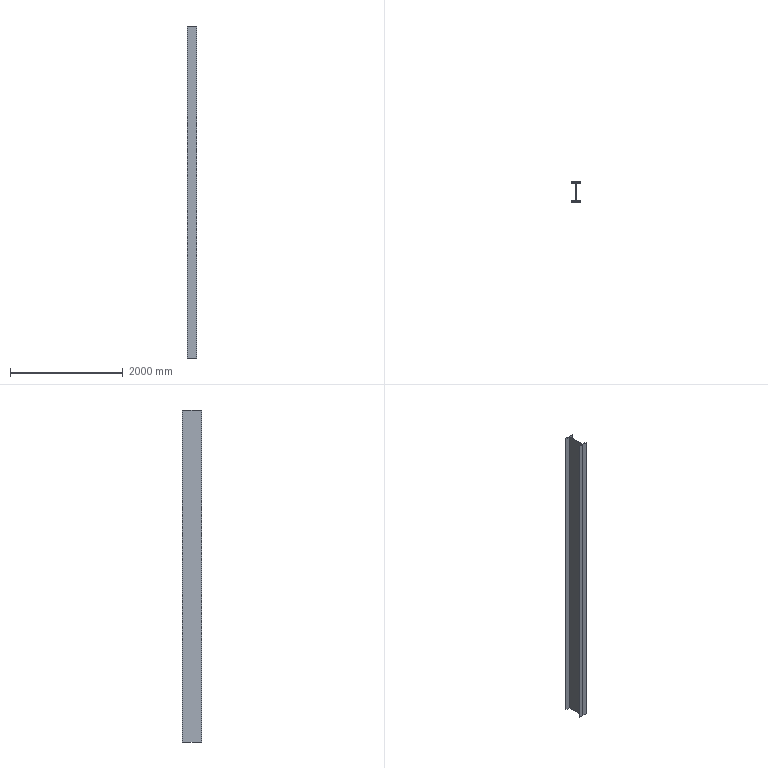Component | NX | ZHIJIA3 | 1 solid | 14 faces | box 175 x 350 x 5900 mm | volume 40120000 mm3 | plane 14
STEP:
#1=CARTESIAN_POINT('',(0.,0.,0.));
#2=DIRECTION('',(0.,0.,1.));
#3=DIRECTION('',(1.,0.,0.));
#4=AXIS2_PLACEMENT_3D('',#1,#2,#3);
#5=CARTESIAN_POINT('',(2412.5,-2965.,800.));
#6=VERTEX_POINT('',#5);
#7=CARTESIAN_POINT('',(2412.5,-2975.,800.));
#8=VERTEX_POINT('',#7);
#9=CARTESIAN_POINT('',(2412.5,-2965.,800.));
#10=DIRECTION('',(-0.,-1.,0.));
#11=VECTOR('',#10,1.);
#12=LINE('',#9,#11);
#13=CARTESIAN_POINT('',(2412.5,-2965.,6700.));
#14=DIRECTION('',(1.,-0.,0.));
#15=DIRECTION('',(0.,1.,0.));
#16=AXIS2_PLACEMENT_3D('',#13,#14,#15);
#17=PLANE('',#16);
#18=CARTESIAN_POINT('',(0.,-5900.));
#19=DIRECTION('',(-1.,0.));
#20=VECTOR('',#19,1.);
#21=LINE('',#18,#20);
#22=(GEOMETRIC_REPRESENTATION_CONTEXT(2)PARAMETRIC_REPRESENTATION_CONTEXT()REPRESENTATION_CONTEXT('',''));
#23=DEFINITIONAL_REPRESENTATION('',(#21),#22);
#24=PCURVE('',#17,#23);
#25=CARTESIAN_POINT('',(2412.5,-2975.,800.));
#26=DIRECTION('',(0.,0.,1.));
#27=DIRECTION('',(1.,0.,0.));
#28=AXIS2_PLACEMENT_3D('',#25,#26,#27);
#29=PLANE('',#28);
#30=CARTESIAN_POINT('',(0.,10.));
#31=DIRECTION('',(-0.,-1.));
#32=VECTOR('',#31,1.);
#33=LINE('',#30,#32);
#34=(GEOMETRIC_REPRESENTATION_CONTEXT(2)PARAMETRIC_REPRESENTATION_CONTEXT()REPRESENTATION_CONTEXT('',''));
#35=DEFINITIONAL_REPRESENTATION('',(#33),#34);
#36=PCURVE('',#29,#35);
#37=SURFACE_CURVE('',#12,(#24,#36),.PCURVE_S1.);
#38=EDGE_CURVE('',#6,#8,#37,.T.);
#39=ORIENTED_EDGE('',*,*,#38,.T.);
#40=CARTESIAN_POINT('',(2412.5,-2975.,6700.));
#41=VERTEX_POINT('',#40);
#42=CARTESIAN_POINT('',(2412.5,-2975.,6700.));
#43=DIRECTION('',(0.,0.,-1.));
#44=VECTOR('',#43,1.);
#45=LINE('',#42,#44);
#46=CARTESIAN_POINT('',(-10.,0.));
#47=DIRECTION('',(0.,-1.));
#48=VECTOR('',#47,1.);
#49=LINE('',#46,#48);
#50=(GEOMETRIC_REPRESENTATION_CONTEXT(2)PARAMETRIC_REPRESENTATION_CONTEXT()REPRESENTATION_CONTEXT('',''));
#51=DEFINITIONAL_REPRESENTATION('',(#49),#50);
#52=PCURVE('',#17,#51);
#53=CARTESIAN_POINT('',(2412.5,-2975.,6700.));
#54=DIRECTION('',(0.,1.,0.));
#55=DIRECTION('',(0.,0.,1.));
#56=AXIS2_PLACEMENT_3D('',#53,#54,#55);
#57=PLANE('',#56);
#58=CARTESIAN_POINT('',(0.,0.));
#59=DIRECTION('',(-1.,0.));
#60=VECTOR('',#59,1.);
#61=LINE('',#58,#60);
#62=(GEOMETRIC_REPRESENTATION_CONTEXT(2)PARAMETRIC_REPRESENTATION_CONTEXT()REPRESENTATION_CONTEXT('',''));
#63=DEFINITIONAL_REPRESENTATION('',(#61),#62);
#64=PCURVE('',#57,#63);
#65=SURFACE_CURVE('',#45,(#52,#64),.PCURVE_S1.);
#66=EDGE_CURVE('',#41,#8,#65,.T.);
#67=ORIENTED_EDGE('',*,*,#66,.F.);
#68=CARTESIAN_POINT('',(2412.5,-2965.,6700.));
#69=VERTEX_POINT('',#68);
#70=CARTESIAN_POINT('',(2412.5,-2965.,6700.));
#71=DIRECTION('',(-0.,-1.,0.));
#72=VECTOR('',#71,1.);
#73=LINE('',#70,#72);
#74=CARTESIAN_POINT('',(0.,0.));
#75=DIRECTION('',(-1.,0.));
#76=VECTOR('',#75,1.);
#77=LINE('',#74,#76);
#78=(GEOMETRIC_REPRESENTATION_CONTEXT(2)PARAMETRIC_REPRESENTATION_CONTEXT()REPRESENTATION_CONTEXT('',''));
#79=DEFINITIONAL_REPRESENTATION('',(#77),#78);
#80=PCURVE('',#17,#79);
#81=CARTESIAN_POINT('',(2412.5,-2975.,6700.));
#82=DIRECTION('',(0.,0.,1.));
#83=DIRECTION('',(1.,0.,0.));
#84=AXIS2_PLACEMENT_3D('',#81,#82,#83);
#85=PLANE('',#84);
#86=CARTESIAN_POINT('',(0.,10.));
#87=DIRECTION('',(-0.,-1.));
#88=VECTOR('',#87,1.);
#89=LINE('',#86,#88);
#90=(GEOMETRIC_REPRESENTATION_CONTEXT(2)PARAMETRIC_REPRESENTATION_CONTEXT()REPRESENTATION_CONTEXT('',''));
#91=DEFINITIONAL_REPRESENTATION('',(#89),#90);
#92=PCURVE('',#85,#91);
#93=SURFACE_CURVE('',#73,(#80,#92),.PCURVE_S1.);
#94=EDGE_CURVE('',#69,#41,#93,.T.);
#95=ORIENTED_EDGE('',*,*,#94,.F.);
#96=CARTESIAN_POINT('',(2412.5,-2965.,6700.));
#97=DIRECTION('',(0.,0.,-1.));
#98=VECTOR('',#97,1.);
#99=LINE('',#96,#98);
#100=CARTESIAN_POINT('',(0.,0.));
#101=DIRECTION('',(0.,-1.));
#102=VECTOR('',#101,1.);
#103=LINE('',#100,#102);
#104=(GEOMETRIC_REPRESENTATION_CONTEXT(2)PARAMETRIC_REPRESENTATION_CONTEXT()REPRESENTATION_CONTEXT('',''));
#105=DEFINITIONAL_REPRESENTATION('',(#103),#104);
#106=PCURVE('',#17,#105);
#107=CARTESIAN_POINT('',(2495.,-2965.,6700.));
#108=DIRECTION('',(0.,-1.,0.));
#109=DIRECTION('',(0.,0.,-1.));
#110=AXIS2_PLACEMENT_3D('',#107,#108,#109);
#111=PLANE('',#110);
#112=CARTESIAN_POINT('',(0.,-82.5));
#113=DIRECTION('',(1.,0.));
#114=VECTOR('',#113,1.);
#115=LINE('',#112,#114);
#116=(GEOMETRIC_REPRESENTATION_CONTEXT(2)PARAMETRIC_REPRESENTATION_CONTEXT()REPRESENTATION_CONTEXT('',''));
#117=DEFINITIONAL_REPRESENTATION('',(#115),#116);
#118=PCURVE('',#111,#117);
#119=SURFACE_CURVE('',#99,(#106,#118),.PCURVE_S1.);
#120=EDGE_CURVE('',#69,#6,#119,.T.);
#121=ORIENTED_EDGE('',*,*,#120,.T.);
#122=EDGE_LOOP('',(#39,#67,#95,#121));
#123=FACE_BOUND('',#122,.T.);
#124=ADVANCED_FACE('',(#123),#17,.F.);
#125=CARTESIAN_POINT('',(2587.5,-2975.,800.));
#126=VERTEX_POINT('',#125);
#127=CARTESIAN_POINT('',(2412.5,-2975.,800.));
#128=DIRECTION('',(1.,0.,0.));
#129=VECTOR('',#128,1.);
#130=LINE('',#127,#129);
#131=CARTESIAN_POINT('',(-5900.,0.));
#132=DIRECTION('',(0.,1.));
#133=VECTOR('',#132,1.);
#134=LINE('',#131,#133);
#135=(GEOMETRIC_REPRESENTATION_CONTEXT(2)PARAMETRIC_REPRESENTATION_CONTEXT()REPRESENTATION_CONTEXT('',''));
#136=DEFINITIONAL_REPRESENTATION('',(#134),#135);
#137=PCURVE('',#57,#136);
#138=CARTESIAN_POINT('',(0.,0.));
#139=DIRECTION('',(1.,0.));
#140=VECTOR('',#139,1.);
#141=LINE('',#138,#140);
#142=(GEOMETRIC_REPRESENTATION_CONTEXT(2)PARAMETRIC_REPRESENTATION_CONTEXT()REPRESENTATION_CONTEXT('',''));
#143=DEFINITIONAL_REPRESENTATION('',(#141),#142);
#144=PCURVE('',#29,#143);
#145=SURFACE_CURVE('',#130,(#137,#144),.PCURVE_S1.);
#146=EDGE_CURVE('',#8,#126,#145,.T.);
#147=ORIENTED_EDGE('',*,*,#146,.T.);
#148=CARTESIAN_POINT('',(2587.5,-2975.,6700.));
#149=VERTEX_POINT('',#148);
#150=CARTESIAN_POINT('',(2587.5,-2975.,6700.));
#151=DIRECTION('',(0.,0.,-1.));
#152=VECTOR('',#151,1.);
#153=LINE('',#150,#152);
#154=CARTESIAN_POINT('',(0.,175.));
#155=DIRECTION('',(-1.,0.));
#156=VECTOR('',#155,1.);
#157=LINE('',#154,#156);
#158=(GEOMETRIC_REPRESENTATION_CONTEXT(2)PARAMETRIC_REPRESENTATION_CONTEXT()REPRESENTATION_CONTEXT('',''));
#159=DEFINITIONAL_REPRESENTATION('',(#157),#158);
#160=PCURVE('',#57,#159);
#161=CARTESIAN_POINT('',(2587.5,-2975.,6700.));
#162=DIRECTION('',(-1.,0.,0.));
#163=DIRECTION('',(-0.,-1.,0.));
#164=AXIS2_PLACEMENT_3D('',#161,#162,#163);
#165=PLANE('',#164);
#166=CARTESIAN_POINT('',(0.,0.));
#167=DIRECTION('',(0.,-1.));
#168=VECTOR('',#167,1.);
#169=LINE('',#166,#168);
#170=(GEOMETRIC_REPRESENTATION_CONTEXT(2)PARAMETRIC_REPRESENTATION_CONTEXT()REPRESENTATION_CONTEXT('',''));
#171=DEFINITIONAL_REPRESENTATION('',(#169),#170);
#172=PCURVE('',#165,#171);
#173=SURFACE_CURVE('',#153,(#160,#172),.PCURVE_S1.);
#174=EDGE_CURVE('',#149,#126,#173,.T.);
#175=ORIENTED_EDGE('',*,*,#174,.F.);
#176=CARTESIAN_POINT('',(2412.5,-2975.,6700.));
#177=DIRECTION('',(1.,0.,0.));
#178=VECTOR('',#177,1.);
#179=LINE('',#176,#178);
#180=CARTESIAN_POINT('',(0.,0.));
#181=DIRECTION('',(0.,1.));
#182=VECTOR('',#181,1.);
#183=LINE('',#180,#182);
#184=(GEOMETRIC_REPRESENTATION_CONTEXT(2)PARAMETRIC_REPRESENTATION_CONTEXT()REPRESENTATION_CONTEXT('',''));
#185=DEFINITIONAL_REPRESENTATION('',(#183),#184);
#186=PCURVE('',#57,#185);
#187=CARTESIAN_POINT('',(0.,0.));
#188=DIRECTION('',(1.,0.));
#189=VECTOR('',#188,1.);
#190=LINE('',#187,#189);
#191=(GEOMETRIC_REPRESENTATION_CONTEXT(2)PARAMETRIC_REPRESENTATION_CONTEXT()REPRESENTATION_CONTEXT('',''));
#192=DEFINITIONAL_REPRESENTATION('',(#190),#191);
#193=PCURVE('',#85,#192);
#194=SURFACE_CURVE('',#179,(#186,#193),.PCURVE_S1.);
#195=EDGE_CURVE('',#41,#149,#194,.T.);
#196=ORIENTED_EDGE('',*,*,#195,.F.);
#197=ORIENTED_EDGE('',*,*,#66,.T.);
#198=EDGE_LOOP('',(#147,#175,#196,#197));
#199=FACE_BOUND('',#198,.T.);
#200=ADVANCED_FACE('',(#199),#57,.F.);
#201=CARTESIAN_POINT('',(2587.5,-2965.,800.));
#202=VERTEX_POINT('',#201);
#203=CARTESIAN_POINT('',(2587.5,-2975.,800.));
#204=DIRECTION('',(0.,1.,0.));
#205=VECTOR('',#204,1.);
#206=LINE('',#203,#205);
#207=CARTESIAN_POINT('',(0.,-5900.));
#208=DIRECTION('',(-1.,0.));
#209=VECTOR('',#208,1.);
#210=LINE('',#207,#209);
#211=(GEOMETRIC_REPRESENTATION_CONTEXT(2)PARAMETRIC_REPRESENTATION_CONTEXT()REPRESENTATION_CONTEXT('',''));
#212=DEFINITIONAL_REPRESENTATION('',(#210),#211);
#213=PCURVE('',#165,#212);
#214=CARTESIAN_POINT('',(175.,0.));
#215=DIRECTION('',(0.,1.));
#216=VECTOR('',#215,1.);
#217=LINE('',#214,#216);
#218=(GEOMETRIC_REPRESENTATION_CONTEXT(2)PARAMETRIC_REPRESENTATION_CONTEXT()REPRESENTATION_CONTEXT('',''));
#219=DEFINITIONAL_REPRESENTATION('',(#217),#218);
#220=PCURVE('',#29,#219);
#221=SURFACE_CURVE('',#206,(#213,#220),.PCURVE_S1.);
#222=EDGE_CURVE('',#126,#202,#221,.T.);
#223=ORIENTED_EDGE('',*,*,#222,.T.);
#224=CARTESIAN_POINT('',(2587.5,-2965.,6700.));
#225=VERTEX_POINT('',#224);
#226=CARTESIAN_POINT('',(2587.5,-2965.,6700.));
#227=DIRECTION('',(0.,0.,-1.));
#228=VECTOR('',#227,1.);
#229=LINE('',#226,#228);
#230=CARTESIAN_POINT('',(-10.,0.));
#231=DIRECTION('',(0.,-1.));
#232=VECTOR('',#231,1.);
#233=LINE('',#230,#232);
#234=(GEOMETRIC_REPRESENTATION_CONTEXT(2)PARAMETRIC_REPRESENTATION_CONTEXT()REPRESENTATION_CONTEXT('',''));
#235=DEFINITIONAL_REPRESENTATION('',(#233),#234);
#236=PCURVE('',#165,#235);
#237=CARTESIAN_POINT('',(2587.5,-2965.,6700.));
#238=DIRECTION('',(0.,-1.,0.));
#239=DIRECTION('',(0.,0.,-1.));
#240=AXIS2_PLACEMENT_3D('',#237,#238,#239);
#241=PLANE('',#240);
#242=CARTESIAN_POINT('',(0.,0.));
#243=DIRECTION('',(1.,0.));
#244=VECTOR('',#243,1.);
#245=LINE('',#242,#244);
#246=(GEOMETRIC_REPRESENTATION_CONTEXT(2)PARAMETRIC_REPRESENTATION_CONTEXT()REPRESENTATION_CONTEXT('',''));
#247=DEFINITIONAL_REPRESENTATION('',(#245),#246);
#248=PCURVE('',#241,#247);
#249=SURFACE_CURVE('',#229,(#236,#248),.PCURVE_S1.);
#250=EDGE_CURVE('',#225,#202,#249,.T.);
#251=ORIENTED_EDGE('',*,*,#250,.F.);
#252=CARTESIAN_POINT('',(2587.5,-2975.,6700.));
#253=DIRECTION('',(0.,1.,0.));
#254=VECTOR('',#253,1.);
#255=LINE('',#252,#254);
#256=CARTESIAN_POINT('',(0.,0.));
#257=DIRECTION('',(-1.,0.));
#258=VECTOR('',#257,1.);
#259=LINE('',#256,#258);
#260=(GEOMETRIC_REPRESENTATION_CONTEXT(2)PARAMETRIC_REPRESENTATION_CONTEXT()REPRESENTATION_CONTEXT('',''));
#261=DEFINITIONAL_REPRESENTATION('',(#259),#260);
#262=PCURVE('',#165,#261);
#263=CARTESIAN_POINT('',(175.,0.));
#264=DIRECTION('',(0.,1.));
#265=VECTOR('',#264,1.);
#266=LINE('',#263,#265);
#267=(GEOMETRIC_REPRESENTATION_CONTEXT(2)PARAMETRIC_REPRESENTATION_CONTEXT()REPRESENTATION_CONTEXT('',''));
#268=DEFINITIONAL_REPRESENTATION('',(#266),#267);
#269=PCURVE('',#85,#268);
#270=SURFACE_CURVE('',#255,(#262,#269),.PCURVE_S1.);
#271=EDGE_CURVE('',#149,#225,#270,.T.);
#272=ORIENTED_EDGE('',*,*,#271,.F.);
#273=ORIENTED_EDGE('',*,*,#174,.T.);
#274=EDGE_LOOP('',(#223,#251,#272,#273));
#275=FACE_BOUND('',#274,.T.);
#276=ADVANCED_FACE('',(#275),#165,.F.);
#277=CARTESIAN_POINT('',(2505.,-2965.,800.));
#278=VERTEX_POINT('',#277);
#279=CARTESIAN_POINT('',(2587.5,-2965.,800.));
#280=DIRECTION('',(-1.,0.,0.));
#281=VECTOR('',#280,1.);
#282=LINE('',#279,#281);
#283=CARTESIAN_POINT('',(5900.,0.));
#284=DIRECTION('',(0.,-1.));
#285=VECTOR('',#284,1.);
#286=LINE('',#283,#285);
#287=(GEOMETRIC_REPRESENTATION_CONTEXT(2)PARAMETRIC_REPRESENTATION_CONTEXT()REPRESENTATION_CONTEXT('',''));
#288=DEFINITIONAL_REPRESENTATION('',(#286),#287);
#289=PCURVE('',#241,#288);
#290=CARTESIAN_POINT('',(175.,10.));
#291=DIRECTION('',(-1.,0.));
#292=VECTOR('',#291,1.);
#293=LINE('',#290,#292);
#294=(GEOMETRIC_REPRESENTATION_CONTEXT(2)PARAMETRIC_REPRESENTATION_CONTEXT()REPRESENTATION_CONTEXT('',''));
#295=DEFINITIONAL_REPRESENTATION('',(#293),#294);
#296=PCURVE('',#29,#295);
#297=SURFACE_CURVE('',#282,(#289,#296),.PCURVE_S1.);
#298=EDGE_CURVE('',#202,#278,#297,.T.);
#299=ORIENTED_EDGE('',*,*,#298,.T.);
#300=CARTESIAN_POINT('',(2505.,-2965.,6700.));
#301=VERTEX_POINT('',#300);
#302=CARTESIAN_POINT('',(2505.,-2965.,6700.));
#303=DIRECTION('',(0.,0.,-1.));
#304=VECTOR('',#303,1.);
#305=LINE('',#302,#304);
#306=CARTESIAN_POINT('',(0.,-82.5));
#307=DIRECTION('',(1.,0.));
#308=VECTOR('',#307,1.);
#309=LINE('',#306,#308);
#310=(GEOMETRIC_REPRESENTATION_CONTEXT(2)PARAMETRIC_REPRESENTATION_CONTEXT()REPRESENTATION_CONTEXT('',''));
#311=DEFINITIONAL_REPRESENTATION('',(#309),#310);
#312=PCURVE('',#241,#311);
#313=CARTESIAN_POINT('',(2505.,-2965.,6700.));
#314=DIRECTION('',(-1.,0.,0.));
#315=DIRECTION('',(-0.,-1.,0.));
#316=AXIS2_PLACEMENT_3D('',#313,#314,#315);
#317=PLANE('',#316);
#318=CARTESIAN_POINT('',(0.,0.));
#319=DIRECTION('',(0.,-1.));
#320=VECTOR('',#319,1.);
#321=LINE('',#318,#320);
#322=(GEOMETRIC_REPRESENTATION_CONTEXT(2)PARAMETRIC_REPRESENTATION_CONTEXT()REPRESENTATION_CONTEXT('',''));
#323=DEFINITIONAL_REPRESENTATION('',(#321),#322);
#324=PCURVE('',#317,#323);
#325=SURFACE_CURVE('',#305,(#312,#324),.PCURVE_S1.);
#326=EDGE_CURVE('',#301,#278,#325,.T.);
#327=ORIENTED_EDGE('',*,*,#326,.F.);
#328=CARTESIAN_POINT('',(2587.5,-2965.,6700.));
#329=DIRECTION('',(-1.,0.,0.));
#330=VECTOR('',#329,1.);
#331=LINE('',#328,#330);
#332=CARTESIAN_POINT('',(0.,0.));
#333=DIRECTION('',(0.,-1.));
#334=VECTOR('',#333,1.);
#335=LINE('',#332,#334);
#336=(GEOMETRIC_REPRESENTATION_CONTEXT(2)PARAMETRIC_REPRESENTATION_CONTEXT()REPRESENTATION_CONTEXT('',''));
#337=DEFINITIONAL_REPRESENTATION('',(#335),#336);
#338=PCURVE('',#241,#337);
#339=CARTESIAN_POINT('',(175.,10.));
#340=DIRECTION('',(-1.,0.));
#341=VECTOR('',#340,1.);
#342=LINE('',#339,#341);
#343=(GEOMETRIC_REPRESENTATION_CONTEXT(2)PARAMETRIC_REPRESENTATION_CONTEXT()REPRESENTATION_CONTEXT('',''));
#344=DEFINITIONAL_REPRESENTATION('',(#342),#343);
#345=PCURVE('',#85,#344);
#346=SURFACE_CURVE('',#331,(#338,#345),.PCURVE_S1.);
#347=EDGE_CURVE('',#225,#301,#346,.T.);
#348=ORIENTED_EDGE('',*,*,#347,.F.);
#349=ORIENTED_EDGE('',*,*,#250,.T.);
#350=EDGE_LOOP('',(#299,#327,#348,#349));
#351=FACE_BOUND('',#350,.T.);
#352=ADVANCED_FACE('',(#351),#241,.F.);
#353=CARTESIAN_POINT('',(2505.,-2635.,800.));
#354=VERTEX_POINT('',#353);
#355=CARTESIAN_POINT('',(2505.,-2965.,800.));
#356=DIRECTION('',(0.,1.,0.));
#357=VECTOR('',#356,1.);
#358=LINE('',#355,#357);
#359=CARTESIAN_POINT('',(0.,-5900.));
#360=DIRECTION('',(-1.,0.));
#361=VECTOR('',#360,1.);
#362=LINE('',#359,#361);
#363=(GEOMETRIC_REPRESENTATION_CONTEXT(2)PARAMETRIC_REPRESENTATION_CONTEXT()REPRESENTATION_CONTEXT('',''));
#364=DEFINITIONAL_REPRESENTATION('',(#362),#363);
#365=PCURVE('',#317,#364);
#366=CARTESIAN_POINT('',(92.5,10.));
#367=DIRECTION('',(0.,1.));
#368=VECTOR('',#367,1.);
#369=LINE('',#366,#368);
#370=(GEOMETRIC_REPRESENTATION_CONTEXT(2)PARAMETRIC_REPRESENTATION_CONTEXT()REPRESENTATION_CONTEXT('',''));
#371=DEFINITIONAL_REPRESENTATION('',(#369),#370);
#372=PCURVE('',#29,#371);
#373=SURFACE_CURVE('',#358,(#365,#372),.PCURVE_S1.);
#374=EDGE_CURVE('',#278,#354,#373,.T.);
#375=ORIENTED_EDGE('',*,*,#374,.T.);
#376=CARTESIAN_POINT('',(2505.,-2635.,6700.));
#377=VERTEX_POINT('',#376);
#378=CARTESIAN_POINT('',(2505.,-2635.,6700.));
#379=DIRECTION('',(0.,0.,-1.));
#380=VECTOR('',#379,1.);
#381=LINE('',#378,#380);
#382=CARTESIAN_POINT('',(-330.,0.));
#383=DIRECTION('',(0.,-1.));
#384=VECTOR('',#383,1.);
#385=LINE('',#382,#384);
#386=(GEOMETRIC_REPRESENTATION_CONTEXT(2)PARAMETRIC_REPRESENTATION_CONTEXT()REPRESENTATION_CONTEXT('',''));
#387=DEFINITIONAL_REPRESENTATION('',(#385),#386);
#388=PCURVE('',#317,#387);
#389=CARTESIAN_POINT('',(2505.,-2635.,6700.));
#390=DIRECTION('',(0.,1.,0.));
#391=DIRECTION('',(0.,0.,1.));
#392=AXIS2_PLACEMENT_3D('',#389,#390,#391);
#393=PLANE('',#392);
#394=CARTESIAN_POINT('',(0.,0.));
#395=DIRECTION('',(-1.,0.));
#396=VECTOR('',#395,1.);
#397=LINE('',#394,#396);
#398=(GEOMETRIC_REPRESENTATION_CONTEXT(2)PARAMETRIC_REPRESENTATION_CONTEXT()REPRESENTATION_CONTEXT('',''));
#399=DEFINITIONAL_REPRESENTATION('',(#397),#398);
#400=PCURVE('',#393,#399);
#401=SURFACE_CURVE('',#381,(#388,#400),.PCURVE_S1.);
#402=EDGE_CURVE('',#377,#354,#401,.T.);
#403=ORIENTED_EDGE('',*,*,#402,.F.);
#404=CARTESIAN_POINT('',(2505.,-2965.,6700.));
#405=DIRECTION('',(0.,1.,0.));
#406=VECTOR('',#405,1.);
#407=LINE('',#404,#406);
#408=CARTESIAN_POINT('',(0.,0.));
#409=DIRECTION('',(-1.,0.));
#410=VECTOR('',#409,1.);
#411=LINE('',#408,#410);
#412=(GEOMETRIC_REPRESENTATION_CONTEXT(2)PARAMETRIC_REPRESENTATION_CONTEXT()REPRESENTATION_CONTEXT('',''));
#413=DEFINITIONAL_REPRESENTATION('',(#411),#412);
#414=PCURVE('',#317,#413);
#415=CARTESIAN_POINT('',(92.5,10.));
#416=DIRECTION('',(0.,1.));
#417=VECTOR('',#416,1.);
#418=LINE('',#415,#417);
#419=(GEOMETRIC_REPRESENTATION_CONTEXT(2)PARAMETRIC_REPRESENTATION_CONTEXT()REPRESENTATION_CONTEXT('',''));
#420=DEFINITIONAL_REPRESENTATION('',(#418),#419);
#421=PCURVE('',#85,#420);
#422=SURFACE_CURVE('',#407,(#414,#421),.PCURVE_S1.);
#423=EDGE_CURVE('',#301,#377,#422,.T.);
#424=ORIENTED_EDGE('',*,*,#423,.F.);
#425=ORIENTED_EDGE('',*,*,#326,.T.);
#426=EDGE_LOOP('',(#375,#403,#424,#425));
#427=FACE_BOUND('',#426,.T.);
#428=ADVANCED_FACE('',(#427),#317,.F.);
#429=CARTESIAN_POINT('',(2587.5,-2635.,800.));
#430=VERTEX_POINT('',#429);
#431=CARTESIAN_POINT('',(2505.,-2635.,800.));
#432=DIRECTION('',(1.,0.,0.));
#433=VECTOR('',#432,1.);
#434=LINE('',#431,#433);
#435=CARTESIAN_POINT('',(-5900.,0.));
#436=DIRECTION('',(0.,1.));
#437=VECTOR('',#436,1.);
#438=LINE('',#435,#437);
#439=(GEOMETRIC_REPRESENTATION_CONTEXT(2)PARAMETRIC_REPRESENTATION_CONTEXT()REPRESENTATION_CONTEXT('',''));
#440=DEFINITIONAL_REPRESENTATION('',(#438),#439);
#441=PCURVE('',#393,#440);
#442=CARTESIAN_POINT('',(92.5,340.));
#443=DIRECTION('',(1.,0.));
#444=VECTOR('',#443,1.);
#445=LINE('',#442,#444);
#446=(GEOMETRIC_REPRESENTATION_CONTEXT(2)PARAMETRIC_REPRESENTATION_CONTEXT()REPRESENTATION_CONTEXT('',''));
#447=DEFINITIONAL_REPRESENTATION('',(#445),#446);
#448=PCURVE('',#29,#447);
#449=SURFACE_CURVE('',#434,(#441,#448),.PCURVE_S1.);
#450=EDGE_CURVE('',#354,#430,#449,.T.);
#451=ORIENTED_EDGE('',*,*,#450,.T.);
#452=CARTESIAN_POINT('',(2587.5,-2635.,6700.));
#453=VERTEX_POINT('',#452);
#454=CARTESIAN_POINT('',(2587.5,-2635.,6700.));
#455=DIRECTION('',(0.,0.,-1.));
#456=VECTOR('',#455,1.);
#457=LINE('',#454,#456);
#458=CARTESIAN_POINT('',(0.,82.5));
#459=DIRECTION('',(-1.,0.));
#460=VECTOR('',#459,1.);
#461=LINE('',#458,#460);
#462=(GEOMETRIC_REPRESENTATION_CONTEXT(2)PARAMETRIC_REPRESENTATION_CONTEXT()REPRESENTATION_CONTEXT('',''));
#463=DEFINITIONAL_REPRESENTATION('',(#461),#462);
#464=PCURVE('',#393,#463);
#465=CARTESIAN_POINT('',(2587.5,-2635.,6700.));
#466=DIRECTION('',(-1.,0.,0.));
#467=DIRECTION('',(-0.,-1.,0.));
#468=AXIS2_PLACEMENT_3D('',#465,#466,#467);
#469=PLANE('',#468);
#470=CARTESIAN_POINT('',(0.,0.));
#471=DIRECTION('',(0.,-1.));
#472=VECTOR('',#471,1.);
#473=LINE('',#470,#472);
#474=(GEOMETRIC_REPRESENTATION_CONTEXT(2)PARAMETRIC_REPRESENTATION_CONTEXT()REPRESENTATION_CONTEXT('',''));
#475=DEFINITIONAL_REPRESENTATION('',(#473),#474);
#476=PCURVE('',#469,#475);
#477=SURFACE_CURVE('',#457,(#464,#476),.PCURVE_S1.);
#478=EDGE_CURVE('',#453,#430,#477,.T.);
#479=ORIENTED_EDGE('',*,*,#478,.F.);
#480=CARTESIAN_POINT('',(2505.,-2635.,6700.));
#481=DIRECTION('',(1.,0.,0.));
#482=VECTOR('',#481,1.);
#483=LINE('',#480,#482);
#484=CARTESIAN_POINT('',(0.,0.));
#485=DIRECTION('',(0.,1.));
#486=VECTOR('',#485,1.);
#487=LINE('',#484,#486);
#488=(GEOMETRIC_REPRESENTATION_CONTEXT(2)PARAMETRIC_REPRESENTATION_CONTEXT()REPRESENTATION_CONTEXT('',''));
#489=DEFINITIONAL_REPRESENTATION('',(#487),#488);
#490=PCURVE('',#393,#489);
#491=CARTESIAN_POINT('',(92.5,340.));
#492=DIRECTION('',(1.,0.));
#493=VECTOR('',#492,1.);
#494=LINE('',#491,#493);
#495=(GEOMETRIC_REPRESENTATION_CONTEXT(2)PARAMETRIC_REPRESENTATION_CONTEXT()REPRESENTATION_CONTEXT('',''));
#496=DEFINITIONAL_REPRESENTATION('',(#494),#495);
#497=PCURVE('',#85,#496);
#498=SURFACE_CURVE('',#483,(#490,#497),.PCURVE_S1.);
#499=EDGE_CURVE('',#377,#453,#498,.T.);
#500=ORIENTED_EDGE('',*,*,#499,.F.);
#501=ORIENTED_EDGE('',*,*,#402,.T.);
#502=EDGE_LOOP('',(#451,#479,#500,#501));
#503=FACE_BOUND('',#502,.T.);
#504=ADVANCED_FACE('',(#503),#393,.F.);
#505=CARTESIAN_POINT('',(2587.5,-2625.,800.));
#506=VERTEX_POINT('',#505);
#507=CARTESIAN_POINT('',(2587.5,-2635.,800.));
#508=DIRECTION('',(0.,1.,0.));
#509=VECTOR('',#508,1.);
#510=LINE('',#507,#509);
#511=CARTESIAN_POINT('',(0.,-5900.));
#512=DIRECTION('',(-1.,0.));
#513=VECTOR('',#512,1.);
#514=LINE('',#511,#513);
#515=(GEOMETRIC_REPRESENTATION_CONTEXT(2)PARAMETRIC_REPRESENTATION_CONTEXT()REPRESENTATION_CONTEXT('',''));
#516=DEFINITIONAL_REPRESENTATION('',(#514),#515);
#517=PCURVE('',#469,#516);
#518=CARTESIAN_POINT('',(175.,340.));
#519=DIRECTION('',(0.,1.));
#520=VECTOR('',#519,1.);
#521=LINE('',#518,#520);
#522=(GEOMETRIC_REPRESENTATION_CONTEXT(2)PARAMETRIC_REPRESENTATION_CONTEXT()REPRESENTATION_CONTEXT('',''));
#523=DEFINITIONAL_REPRESENTATION('',(#521),#522);
#524=PCURVE('',#29,#523);
#525=SURFACE_CURVE('',#510,(#517,#524),.PCURVE_S1.);
#526=EDGE_CURVE('',#430,#506,#525,.T.);
#527=ORIENTED_EDGE('',*,*,#526,.T.);
#528=CARTESIAN_POINT('',(2587.5,-2625.,6700.));
#529=VERTEX_POINT('',#528);
#530=CARTESIAN_POINT('',(2587.5,-2625.,6700.));
#531=DIRECTION('',(0.,0.,-1.));
#532=VECTOR('',#531,1.);
#533=LINE('',#530,#532);
#534=CARTESIAN_POINT('',(-10.,0.));
#535=DIRECTION('',(0.,-1.));
#536=VECTOR('',#535,1.);
#537=LINE('',#534,#536);
#538=(GEOMETRIC_REPRESENTATION_CONTEXT(2)PARAMETRIC_REPRESENTATION_CONTEXT()REPRESENTATION_CONTEXT('',''));
#539=DEFINITIONAL_REPRESENTATION('',(#537),#538);
#540=PCURVE('',#469,#539);
#541=CARTESIAN_POINT('',(2587.5,-2625.,6700.));
#542=DIRECTION('',(0.,-1.,0.));
#543=DIRECTION('',(0.,0.,-1.));
#544=AXIS2_PLACEMENT_3D('',#541,#542,#543);
#545=PLANE('',#544);
#546=CARTESIAN_POINT('',(0.,0.));
#547=DIRECTION('',(1.,0.));
#548=VECTOR('',#547,1.);
#549=LINE('',#546,#548);
#550=(GEOMETRIC_REPRESENTATION_CONTEXT(2)PARAMETRIC_REPRESENTATION_CONTEXT()REPRESENTATION_CONTEXT('',''));
#551=DEFINITIONAL_REPRESENTATION('',(#549),#550);
#552=PCURVE('',#545,#551);
#553=SURFACE_CURVE('',#533,(#540,#552),.PCURVE_S1.);
#554=EDGE_CURVE('',#529,#506,#553,.T.);
#555=ORIENTED_EDGE('',*,*,#554,.F.);
#556=CARTESIAN_POINT('',(2587.5,-2635.,6700.));
#557=DIRECTION('',(0.,1.,0.));
#558=VECTOR('',#557,1.);
#559=LINE('',#556,#558);
#560=CARTESIAN_POINT('',(0.,0.));
#561=DIRECTION('',(-1.,0.));
#562=VECTOR('',#561,1.);
#563=LINE('',#560,#562);
#564=(GEOMETRIC_REPRESENTATION_CONTEXT(2)PARAMETRIC_REPRESENTATION_CONTEXT()REPRESENTATION_CONTEXT('',''));
#565=DEFINITIONAL_REPRESENTATION('',(#563),#564);
#566=PCURVE('',#469,#565);
#567=CARTESIAN_POINT('',(175.,340.));
#568=DIRECTION('',(0.,1.));
#569=VECTOR('',#568,1.);
#570=LINE('',#567,#569);
#571=(GEOMETRIC_REPRESENTATION_CONTEXT(2)PARAMETRIC_REPRESENTATION_CONTEXT()REPRESENTATION_CONTEXT('',''));
#572=DEFINITIONAL_REPRESENTATION('',(#570),#571);
#573=PCURVE('',#85,#572);
#574=SURFACE_CURVE('',#559,(#566,#573),.PCURVE_S1.);
#575=EDGE_CURVE('',#453,#529,#574,.T.);
#576=ORIENTED_EDGE('',*,*,#575,.F.);
#577=ORIENTED_EDGE('',*,*,#478,.T.);
#578=EDGE_LOOP('',(#527,#555,#576,#577));
#579=FACE_BOUND('',#578,.T.);
#580=ADVANCED_FACE('',(#579),#469,.F.);
#581=CARTESIAN_POINT('',(2412.5,-2625.,800.));
#582=VERTEX_POINT('',#581);
#583=CARTESIAN_POINT('',(2587.5,-2625.,800.));
#584=DIRECTION('',(-1.,0.,0.));
#585=VECTOR('',#584,1.);
#586=LINE('',#583,#585);
#587=CARTESIAN_POINT('',(5900.,0.));
#588=DIRECTION('',(0.,-1.));
#589=VECTOR('',#588,1.);
#590=LINE('',#587,#589);
#591=(GEOMETRIC_REPRESENTATION_CONTEXT(2)PARAMETRIC_REPRESENTATION_CONTEXT()REPRESENTATION_CONTEXT('',''));
#592=DEFINITIONAL_REPRESENTATION('',(#590),#591);
#593=PCURVE('',#545,#592);
#594=CARTESIAN_POINT('',(175.,350.));
#595=DIRECTION('',(-1.,0.));
#596=VECTOR('',#595,1.);
#597=LINE('',#594,#596);
#598=(GEOMETRIC_REPRESENTATION_CONTEXT(2)PARAMETRIC_REPRESENTATION_CONTEXT()REPRESENTATION_CONTEXT('',''));
#599=DEFINITIONAL_REPRESENTATION('',(#597),#598);
#600=PCURVE('',#29,#599);
#601=SURFACE_CURVE('',#586,(#593,#600),.PCURVE_S1.);
#602=EDGE_CURVE('',#506,#582,#601,.T.);
#603=ORIENTED_EDGE('',*,*,#602,.T.);
#604=CARTESIAN_POINT('',(2412.5,-2625.,6700.));
#605=VERTEX_POINT('',#604);
#606=CARTESIAN_POINT('',(2412.5,-2625.,6700.));
#607=DIRECTION('',(0.,0.,-1.));
#608=VECTOR('',#607,1.);
#609=LINE('',#606,#608);
#610=CARTESIAN_POINT('',(0.,-175.));
#611=DIRECTION('',(1.,0.));
#612=VECTOR('',#611,1.);
#613=LINE('',#610,#612);
#614=(GEOMETRIC_REPRESENTATION_CONTEXT(2)PARAMETRIC_REPRESENTATION_CONTEXT()REPRESENTATION_CONTEXT('',''));
#615=DEFINITIONAL_REPRESENTATION('',(#613),#614);
#616=PCURVE('',#545,#615);
#617=CARTESIAN_POINT('',(2412.5,-2625.,6700.));
#618=DIRECTION('',(1.,-0.,0.));
#619=DIRECTION('',(0.,1.,0.));
#620=AXIS2_PLACEMENT_3D('',#617,#618,#619);
#621=PLANE('',#620);
#622=CARTESIAN_POINT('',(0.,0.));
#623=DIRECTION('',(0.,-1.));
#624=VECTOR('',#623,1.);
#625=LINE('',#622,#624);
#626=(GEOMETRIC_REPRESENTATION_CONTEXT(2)PARAMETRIC_REPRESENTATION_CONTEXT()REPRESENTATION_CONTEXT('',''));
#627=DEFINITIONAL_REPRESENTATION('',(#625),#626);
#628=PCURVE('',#621,#627);
#629=SURFACE_CURVE('',#609,(#616,#628),.PCURVE_S1.);
#630=EDGE_CURVE('',#605,#582,#629,.T.);
#631=ORIENTED_EDGE('',*,*,#630,.F.);
#632=CARTESIAN_POINT('',(2587.5,-2625.,6700.));
#633=DIRECTION('',(-1.,0.,0.));
#634=VECTOR('',#633,1.);
#635=LINE('',#632,#634);
#636=CARTESIAN_POINT('',(0.,0.));
#637=DIRECTION('',(0.,-1.));
#638=VECTOR('',#637,1.);
#639=LINE('',#636,#638);
#640=(GEOMETRIC_REPRESENTATION_CONTEXT(2)PARAMETRIC_REPRESENTATION_CONTEXT()REPRESENTATION_CONTEXT('',''));
#641=DEFINITIONAL_REPRESENTATION('',(#639),#640);
#642=PCURVE('',#545,#641);
#643=CARTESIAN_POINT('',(175.,350.));
#644=DIRECTION('',(-1.,0.));
#645=VECTOR('',#644,1.);
#646=LINE('',#643,#645);
#647=(GEOMETRIC_REPRESENTATION_CONTEXT(2)PARAMETRIC_REPRESENTATION_CONTEXT()REPRESENTATION_CONTEXT('',''));
#648=DEFINITIONAL_REPRESENTATION('',(#646),#647);
#649=PCURVE('',#85,#648);
#650=SURFACE_CURVE('',#635,(#642,#649),.PCURVE_S1.);
#651=EDGE_CURVE('',#529,#605,#650,.T.);
#652=ORIENTED_EDGE('',*,*,#651,.F.);
#653=ORIENTED_EDGE('',*,*,#554,.T.);
#654=EDGE_LOOP('',(#603,#631,#652,#653));
#655=FACE_BOUND('',#654,.T.);
#656=ADVANCED_FACE('',(#655),#545,.F.);
#657=CARTESIAN_POINT('',(2412.5,-2635.,800.));
#658=VERTEX_POINT('',#657);
#659=CARTESIAN_POINT('',(2412.5,-2625.,800.));
#660=DIRECTION('',(-0.,-1.,0.));
#661=VECTOR('',#660,1.);
#662=LINE('',#659,#661);
#663=CARTESIAN_POINT('',(0.,-5900.));
#664=DIRECTION('',(-1.,0.));
#665=VECTOR('',#664,1.);
#666=LINE('',#663,#665);
#667=(GEOMETRIC_REPRESENTATION_CONTEXT(2)PARAMETRIC_REPRESENTATION_CONTEXT()REPRESENTATION_CONTEXT('',''));
#668=DEFINITIONAL_REPRESENTATION('',(#666),#667);
#669=PCURVE('',#621,#668);
#670=CARTESIAN_POINT('',(0.,350.));
#671=DIRECTION('',(-0.,-1.));
#672=VECTOR('',#671,1.);
#673=LINE('',#670,#672);
#674=(GEOMETRIC_REPRESENTATION_CONTEXT(2)PARAMETRIC_REPRESENTATION_CONTEXT()REPRESENTATION_CONTEXT('',''));
#675=DEFINITIONAL_REPRESENTATION('',(#673),#674);
#676=PCURVE('',#29,#675);
#677=SURFACE_CURVE('',#662,(#669,#676),.PCURVE_S1.);
#678=EDGE_CURVE('',#582,#658,#677,.T.);
#679=ORIENTED_EDGE('',*,*,#678,.T.);
#680=CARTESIAN_POINT('',(2412.5,-2635.,6700.));
#681=VERTEX_POINT('',#680);
#682=CARTESIAN_POINT('',(2412.5,-2635.,6700.));
#683=DIRECTION('',(0.,0.,-1.));
#684=VECTOR('',#683,1.);
#685=LINE('',#682,#684);
#686=CARTESIAN_POINT('',(-10.,0.));
#687=DIRECTION('',(0.,-1.));
#688=VECTOR('',#687,1.);
#689=LINE('',#686,#688);
#690=(GEOMETRIC_REPRESENTATION_CONTEXT(2)PARAMETRIC_REPRESENTATION_CONTEXT()REPRESENTATION_CONTEXT('',''));
#691=DEFINITIONAL_REPRESENTATION('',(#689),#690);
#692=PCURVE('',#621,#691);
#693=CARTESIAN_POINT('',(2412.5,-2635.,6700.));
#694=DIRECTION('',(0.,1.,0.));
#695=DIRECTION('',(0.,0.,1.));
#696=AXIS2_PLACEMENT_3D('',#693,#694,#695);
#697=PLANE('',#696);
#698=CARTESIAN_POINT('',(0.,0.));
#699=DIRECTION('',(-1.,0.));
#700=VECTOR('',#699,1.);
#701=LINE('',#698,#700);
#702=(GEOMETRIC_REPRESENTATION_CONTEXT(2)PARAMETRIC_REPRESENTATION_CONTEXT()REPRESENTATION_CONTEXT('',''));
#703=DEFINITIONAL_REPRESENTATION('',(#701),#702);
#704=PCURVE('',#697,#703);
#705=SURFACE_CURVE('',#685,(#692,#704),.PCURVE_S1.);
#706=EDGE_CURVE('',#681,#658,#705,.T.);
#707=ORIENTED_EDGE('',*,*,#706,.F.);
#708=CARTESIAN_POINT('',(2412.5,-2625.,6700.));
#709=DIRECTION('',(-0.,-1.,0.));
#710=VECTOR('',#709,1.);
#711=LINE('',#708,#710);
#712=CARTESIAN_POINT('',(0.,0.));
#713=DIRECTION('',(-1.,0.));
#714=VECTOR('',#713,1.);
#715=LINE('',#712,#714);
#716=(GEOMETRIC_REPRESENTATION_CONTEXT(2)PARAMETRIC_REPRESENTATION_CONTEXT()REPRESENTATION_CONTEXT('',''));
#717=DEFINITIONAL_REPRESENTATION('',(#715),#716);
#718=PCURVE('',#621,#717);
#719=CARTESIAN_POINT('',(0.,350.));
#720=DIRECTION('',(-0.,-1.));
#721=VECTOR('',#720,1.);
#722=LINE('',#719,#721);
#723=(GEOMETRIC_REPRESENTATION_CONTEXT(2)PARAMETRIC_REPRESENTATION_CONTEXT()REPRESENTATION_CONTEXT('',''));
#724=DEFINITIONAL_REPRESENTATION('',(#722),#723);
#725=PCURVE('',#85,#724);
#726=SURFACE_CURVE('',#711,(#718,#725),.PCURVE_S1.);
#727=EDGE_CURVE('',#605,#681,#726,.T.);
#728=ORIENTED_EDGE('',*,*,#727,.F.);
#729=ORIENTED_EDGE('',*,*,#630,.T.);
#730=EDGE_LOOP('',(#679,#707,#728,#729));
#731=FACE_BOUND('',#730,.T.);
#732=ADVANCED_FACE('',(#731),#621,.F.);
#733=CARTESIAN_POINT('',(2495.,-2635.,800.));
#734=VERTEX_POINT('',#733);
#735=CARTESIAN_POINT('',(2412.5,-2635.,800.));
#736=DIRECTION('',(1.,0.,0.));
#737=VECTOR('',#736,1.);
#738=LINE('',#735,#737);
#739=CARTESIAN_POINT('',(-5900.,0.));
#740=DIRECTION('',(0.,1.));
#741=VECTOR('',#740,1.);
#742=LINE('',#739,#741);
#743=(GEOMETRIC_REPRESENTATION_CONTEXT(2)PARAMETRIC_REPRESENTATION_CONTEXT()REPRESENTATION_CONTEXT('',''));
#744=DEFINITIONAL_REPRESENTATION('',(#742),#743);
#745=PCURVE('',#697,#744);
#746=CARTESIAN_POINT('',(0.,340.));
#747=DIRECTION('',(1.,0.));
#748=VECTOR('',#747,1.);
#749=LINE('',#746,#748);
#750=(GEOMETRIC_REPRESENTATION_CONTEXT(2)PARAMETRIC_REPRESENTATION_CONTEXT()REPRESENTATION_CONTEXT('',''));
#751=DEFINITIONAL_REPRESENTATION('',(#749),#750);
#752=PCURVE('',#29,#751);
#753=SURFACE_CURVE('',#738,(#745,#752),.PCURVE_S1.);
#754=EDGE_CURVE('',#658,#734,#753,.T.);
#755=ORIENTED_EDGE('',*,*,#754,.T.);
#756=CARTESIAN_POINT('',(2495.,-2635.,6700.));
#757=VERTEX_POINT('',#756);
#758=CARTESIAN_POINT('',(2495.,-2635.,6700.));
#759=DIRECTION('',(0.,0.,-1.));
#760=VECTOR('',#759,1.);
#761=LINE('',#758,#760);
#762=CARTESIAN_POINT('',(0.,82.5));
#763=DIRECTION('',(-1.,0.));
#764=VECTOR('',#763,1.);
#765=LINE('',#762,#764);
#766=(GEOMETRIC_REPRESENTATION_CONTEXT(2)PARAMETRIC_REPRESENTATION_CONTEXT()REPRESENTATION_CONTEXT('',''));
#767=DEFINITIONAL_REPRESENTATION('',(#765),#766);
#768=PCURVE('',#697,#767);
#769=CARTESIAN_POINT('',(2495.,-2635.,6700.));
#770=DIRECTION('',(1.,-0.,0.));
#771=DIRECTION('',(0.,1.,0.));
#772=AXIS2_PLACEMENT_3D('',#769,#770,#771);
#773=PLANE('',#772);
#774=CARTESIAN_POINT('',(0.,0.));
#775=DIRECTION('',(0.,-1.));
#776=VECTOR('',#775,1.);
#777=LINE('',#774,#776);
#778=(GEOMETRIC_REPRESENTATION_CONTEXT(2)PARAMETRIC_REPRESENTATION_CONTEXT()REPRESENTATION_CONTEXT('',''));
#779=DEFINITIONAL_REPRESENTATION('',(#777),#778);
#780=PCURVE('',#773,#779);
#781=SURFACE_CURVE('',#761,(#768,#780),.PCURVE_S1.);
#782=EDGE_CURVE('',#757,#734,#781,.T.);
#783=ORIENTED_EDGE('',*,*,#782,.F.);
#784=CARTESIAN_POINT('',(2412.5,-2635.,6700.));
#785=DIRECTION('',(1.,0.,0.));
#786=VECTOR('',#785,1.);
#787=LINE('',#784,#786);
#788=CARTESIAN_POINT('',(0.,0.));
#789=DIRECTION('',(0.,1.));
#790=VECTOR('',#789,1.);
#791=LINE('',#788,#790);
#792=(GEOMETRIC_REPRESENTATION_CONTEXT(2)PARAMETRIC_REPRESENTATION_CONTEXT()REPRESENTATION_CONTEXT('',''));
#793=DEFINITIONAL_REPRESENTATION('',(#791),#792);
#794=PCURVE('',#697,#793);
#795=CARTESIAN_POINT('',(0.,340.));
#796=DIRECTION('',(1.,0.));
#797=VECTOR('',#796,1.);
#798=LINE('',#795,#797);
#799=(GEOMETRIC_REPRESENTATION_CONTEXT(2)PARAMETRIC_REPRESENTATION_CONTEXT()REPRESENTATION_CONTEXT('',''));
#800=DEFINITIONAL_REPRESENTATION('',(#798),#799);
#801=PCURVE('',#85,#800);
#802=SURFACE_CURVE('',#787,(#794,#801),.PCURVE_S1.);
#803=EDGE_CURVE('',#681,#757,#802,.T.);
#804=ORIENTED_EDGE('',*,*,#803,.F.);
#805=ORIENTED_EDGE('',*,*,#706,.T.);
#806=EDGE_LOOP('',(#755,#783,#804,#805));
#807=FACE_BOUND('',#806,.T.);
#808=ADVANCED_FACE('',(#807),#697,.F.);
#809=CARTESIAN_POINT('',(2495.,-2965.,800.));
#810=VERTEX_POINT('',#809);
#811=CARTESIAN_POINT('',(2495.,-2635.,800.));
#812=DIRECTION('',(-0.,-1.,0.));
#813=VECTOR('',#812,1.);
#814=LINE('',#811,#813);
#815=CARTESIAN_POINT('',(0.,-5900.));
#816=DIRECTION('',(-1.,0.));
#817=VECTOR('',#816,1.);
#818=LINE('',#815,#817);
#819=(GEOMETRIC_REPRESENTATION_CONTEXT(2)PARAMETRIC_REPRESENTATION_CONTEXT()REPRESENTATION_CONTEXT('',''));
#820=DEFINITIONAL_REPRESENTATION('',(#818),#819);
#821=PCURVE('',#773,#820);
#822=CARTESIAN_POINT('',(82.5,340.));
#823=DIRECTION('',(-0.,-1.));
#824=VECTOR('',#823,1.);
#825=LINE('',#822,#824);
#826=(GEOMETRIC_REPRESENTATION_CONTEXT(2)PARAMETRIC_REPRESENTATION_CONTEXT()REPRESENTATION_CONTEXT('',''));
#827=DEFINITIONAL_REPRESENTATION('',(#825),#826);
#828=PCURVE('',#29,#827);
#829=SURFACE_CURVE('',#814,(#821,#828),.PCURVE_S1.);
#830=EDGE_CURVE('',#734,#810,#829,.T.);
#831=ORIENTED_EDGE('',*,*,#830,.T.);
#832=CARTESIAN_POINT('',(2495.,-2965.,6700.));
#833=VERTEX_POINT('',#832);
#834=CARTESIAN_POINT('',(2495.,-2965.,6700.));
#835=DIRECTION('',(0.,0.,-1.));
#836=VECTOR('',#835,1.);
#837=LINE('',#834,#836);
#838=CARTESIAN_POINT('',(-330.,0.));
#839=DIRECTION('',(0.,-1.));
#840=VECTOR('',#839,1.);
#841=LINE('',#838,#840);
#842=(GEOMETRIC_REPRESENTATION_CONTEXT(2)PARAMETRIC_REPRESENTATION_CONTEXT()REPRESENTATION_CONTEXT('',''));
#843=DEFINITIONAL_REPRESENTATION('',(#841),#842);
#844=PCURVE('',#773,#843);
#845=CARTESIAN_POINT('',(0.,0.));
#846=DIRECTION('',(1.,0.));
#847=VECTOR('',#846,1.);
#848=LINE('',#845,#847);
#849=(GEOMETRIC_REPRESENTATION_CONTEXT(2)PARAMETRIC_REPRESENTATION_CONTEXT()REPRESENTATION_CONTEXT('',''));
#850=DEFINITIONAL_REPRESENTATION('',(#848),#849);
#851=PCURVE('',#111,#850);
#852=SURFACE_CURVE('',#837,(#844,#851),.PCURVE_S1.);
#853=EDGE_CURVE('',#833,#810,#852,.T.);
#854=ORIENTED_EDGE('',*,*,#853,.F.);
#855=CARTESIAN_POINT('',(2495.,-2635.,6700.));
#856=DIRECTION('',(-0.,-1.,0.));
#857=VECTOR('',#856,1.);
#858=LINE('',#855,#857);
#859=CARTESIAN_POINT('',(0.,0.));
#860=DIRECTION('',(-1.,0.));
#861=VECTOR('',#860,1.);
#862=LINE('',#859,#861);
#863=(GEOMETRIC_REPRESENTATION_CONTEXT(2)PARAMETRIC_REPRESENTATION_CONTEXT()REPRESENTATION_CONTEXT('',''));
#864=DEFINITIONAL_REPRESENTATION('',(#862),#863);
#865=PCURVE('',#773,#864);
#866=CARTESIAN_POINT('',(82.5,340.));
#867=DIRECTION('',(-0.,-1.));
#868=VECTOR('',#867,1.);
#869=LINE('',#866,#868);
#870=(GEOMETRIC_REPRESENTATION_CONTEXT(2)PARAMETRIC_REPRESENTATION_CONTEXT()REPRESENTATION_CONTEXT('',''));
#871=DEFINITIONAL_REPRESENTATION('',(#869),#870);
#872=PCURVE('',#85,#871);
#873=SURFACE_CURVE('',#858,(#865,#872),.PCURVE_S1.);
#874=EDGE_CURVE('',#757,#833,#873,.T.);
#875=ORIENTED_EDGE('',*,*,#874,.F.);
#876=ORIENTED_EDGE('',*,*,#782,.T.);
#877=EDGE_LOOP('',(#831,#854,#875,#876));
#878=FACE_BOUND('',#877,.T.);
#879=ADVANCED_FACE('',(#878),#773,.F.);
#880=CARTESIAN_POINT('',(2495.,-2965.,800.));
#881=DIRECTION('',(-1.,0.,0.));
#882=VECTOR('',#881,1.);
#883=LINE('',#880,#882);
#884=CARTESIAN_POINT('',(5900.,0.));
#885=DIRECTION('',(0.,-1.));
#886=VECTOR('',#885,1.);
#887=LINE('',#884,#886);
#888=(GEOMETRIC_REPRESENTATION_CONTEXT(2)PARAMETRIC_REPRESENTATION_CONTEXT()REPRESENTATION_CONTEXT('',''));
#889=DEFINITIONAL_REPRESENTATION('',(#887),#888);
#890=PCURVE('',#111,#889);
#891=CARTESIAN_POINT('',(82.5,10.));
#892=DIRECTION('',(-1.,0.));
#893=VECTOR('',#892,1.);
#894=LINE('',#891,#893);
#895=(GEOMETRIC_REPRESENTATION_CONTEXT(2)PARAMETRIC_REPRESENTATION_CONTEXT()REPRESENTATION_CONTEXT('',''));
#896=DEFINITIONAL_REPRESENTATION('',(#894),#895);
#897=PCURVE('',#29,#896);
#898=SURFACE_CURVE('',#883,(#890,#897),.PCURVE_S1.);
#899=EDGE_CURVE('',#810,#6,#898,.T.);
#900=ORIENTED_EDGE('',*,*,#899,.T.);
#901=ORIENTED_EDGE('',*,*,#120,.F.);
#902=CARTESIAN_POINT('',(2495.,-2965.,6700.));
#903=DIRECTION('',(-1.,0.,0.));
#904=VECTOR('',#903,1.);
#905=LINE('',#902,#904);
#906=CARTESIAN_POINT('',(0.,0.));
#907=DIRECTION('',(0.,-1.));
#908=VECTOR('',#907,1.);
#909=LINE('',#906,#908);
#910=(GEOMETRIC_REPRESENTATION_CONTEXT(2)PARAMETRIC_REPRESENTATION_CONTEXT()REPRESENTATION_CONTEXT('',''));
#911=DEFINITIONAL_REPRESENTATION('',(#909),#910);
#912=PCURVE('',#111,#911);
#913=CARTESIAN_POINT('',(82.5,10.));
#914=DIRECTION('',(-1.,0.));
#915=VECTOR('',#914,1.);
#916=LINE('',#913,#915);
#917=(GEOMETRIC_REPRESENTATION_CONTEXT(2)PARAMETRIC_REPRESENTATION_CONTEXT()REPRESENTATION_CONTEXT('',''));
#918=DEFINITIONAL_REPRESENTATION('',(#916),#917);
#919=PCURVE('',#85,#918);
#920=SURFACE_CURVE('',#905,(#912,#919),.PCURVE_S1.);
#921=EDGE_CURVE('',#833,#69,#920,.T.);
#922=ORIENTED_EDGE('',*,*,#921,.F.);
#923=ORIENTED_EDGE('',*,*,#853,.T.);
#924=EDGE_LOOP('',(#900,#901,#922,#923));
#925=FACE_BOUND('',#924,.T.);
#926=ADVANCED_FACE('',(#925),#111,.F.);
#927=ORIENTED_EDGE('',*,*,#94,.T.);
#928=ORIENTED_EDGE('',*,*,#195,.T.);
#929=ORIENTED_EDGE('',*,*,#271,.T.);
#930=ORIENTED_EDGE('',*,*,#347,.T.);
#931=ORIENTED_EDGE('',*,*,#423,.T.);
#932=ORIENTED_EDGE('',*,*,#499,.T.);
#933=ORIENTED_EDGE('',*,*,#575,.T.);
#934=ORIENTED_EDGE('',*,*,#651,.T.);
#935=ORIENTED_EDGE('',*,*,#727,.T.);
#936=ORIENTED_EDGE('',*,*,#803,.T.);
#937=ORIENTED_EDGE('',*,*,#874,.T.);
#938=ORIENTED_EDGE('',*,*,#921,.T.);
#939=EDGE_LOOP('',(#927,#928,#929,#930,#931,#932,#933,#934,#935,#936,#937,#938));
#940=FACE_BOUND('',#939,.T.);
#941=ADVANCED_FACE('',(#940),#85,.T.);
#942=ORIENTED_EDGE('',*,*,#38,.F.);
#943=ORIENTED_EDGE('',*,*,#899,.F.);
#944=ORIENTED_EDGE('',*,*,#830,.F.);
#945=ORIENTED_EDGE('',*,*,#754,.F.);
#946=ORIENTED_EDGE('',*,*,#678,.F.);
#947=ORIENTED_EDGE('',*,*,#602,.F.);
#948=ORIENTED_EDGE('',*,*,#526,.F.);
#949=ORIENTED_EDGE('',*,*,#450,.F.);
#950=ORIENTED_EDGE('',*,*,#374,.F.);
#951=ORIENTED_EDGE('',*,*,#298,.F.);
#952=ORIENTED_EDGE('',*,*,#222,.F.);
#953=ORIENTED_EDGE('',*,*,#146,.F.);
#954=EDGE_LOOP('',(#942,#943,#944,#945,#946,#947,#948,#949,#950,#951,#952,#953));
#955=FACE_BOUND('',#954,.T.);
#956=ADVANCED_FACE('',(#955),#29,.F.);
#957=CLOSED_SHELL('',(#124,#200,#276,#352,#428,#504,#580,#656,#732,#808,#879,#926,#941,#956));
#958=MANIFOLD_SOLID_BREP('',#957);
#959=(LENGTH_UNIT()NAMED_UNIT(*)SI_UNIT(.MILLI.,.METRE.));
#960=UNCERTAINTY_MEASURE_WITH_UNIT(LENGTH_MEASURE(0.0000001),#959,'','');
#961=(NAMED_UNIT(*)PLANE_ANGLE_UNIT()SI_UNIT($,.RADIAN.));
#962=(NAMED_UNIT(*)SI_UNIT($,.STERADIAN.)SOLID_ANGLE_UNIT());
#963=(GEOMETRIC_REPRESENTATION_CONTEXT(3)GLOBAL_UNCERTAINTY_ASSIGNED_CONTEXT((#960))GLOBAL_UNIT_ASSIGNED_CONTEXT((#959,#961,#962))REPRESENTATION_CONTEXT('',''));
#964=ADVANCED_BREP_SHAPE_REPRESENTATION('',(#4,#958),#963);